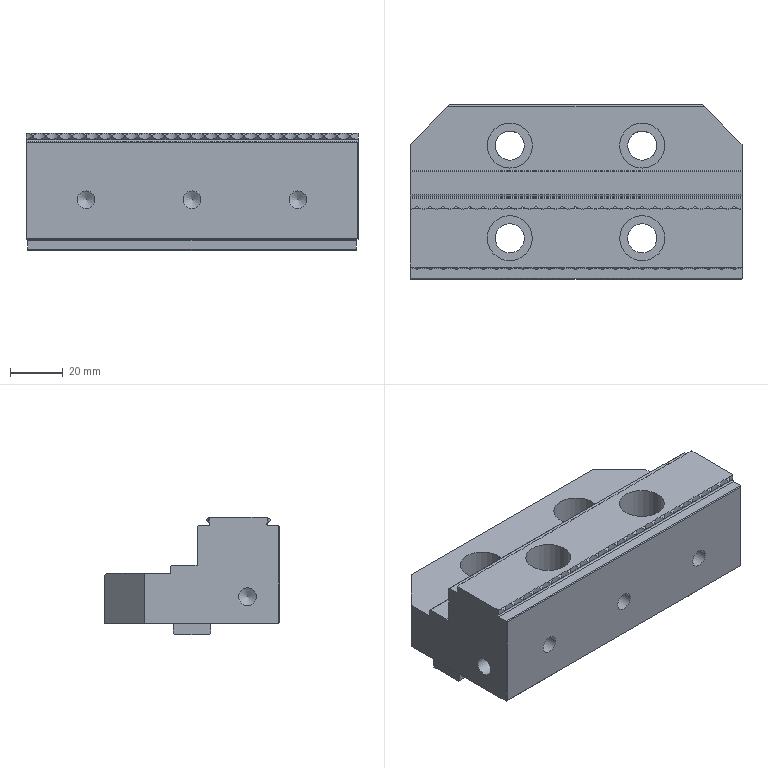Component | NX | JAW_FIXED_125 | 1 solid | 281 faces | volume 219035 mm3 | plane 195 | cylinder 81 | cone 5 | commonest cylinder face diameters 6 x52 12 x5 11 x4 17 x4 4 x4 1 x3 6.65 x3 6.8 x2